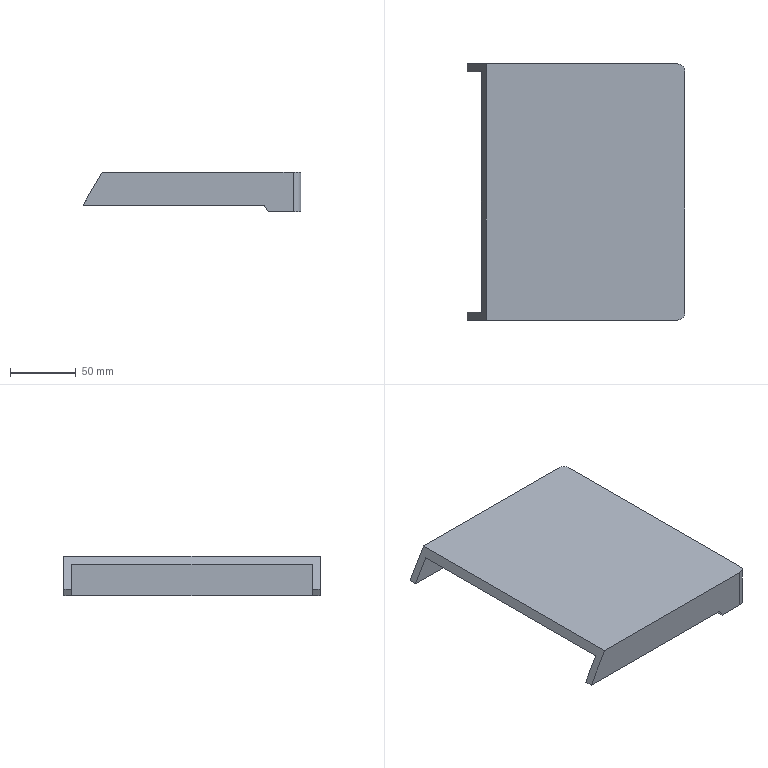Component | NX | SLIDE_COVER_SMALL | 1 solid | 20 faces | volume 242217 mm3 | plane 16 | cylinder 4 | commonest cylinder face diameters 12 x2 3 x2